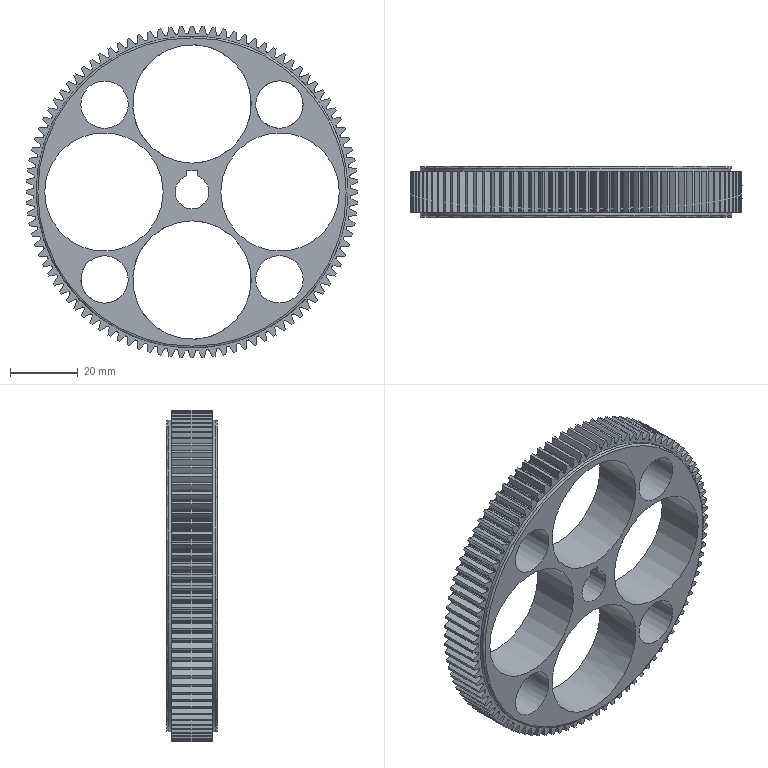Component | NX | BIG_GEAR | 1 solid | 596 faces | volume 38340 mm3 | other 480 | cylinder 107 | plane 7 | torus 2 | commonest cylinder face diameters 93.5 x96 14 x4 35 x4 92 x2 10 x1